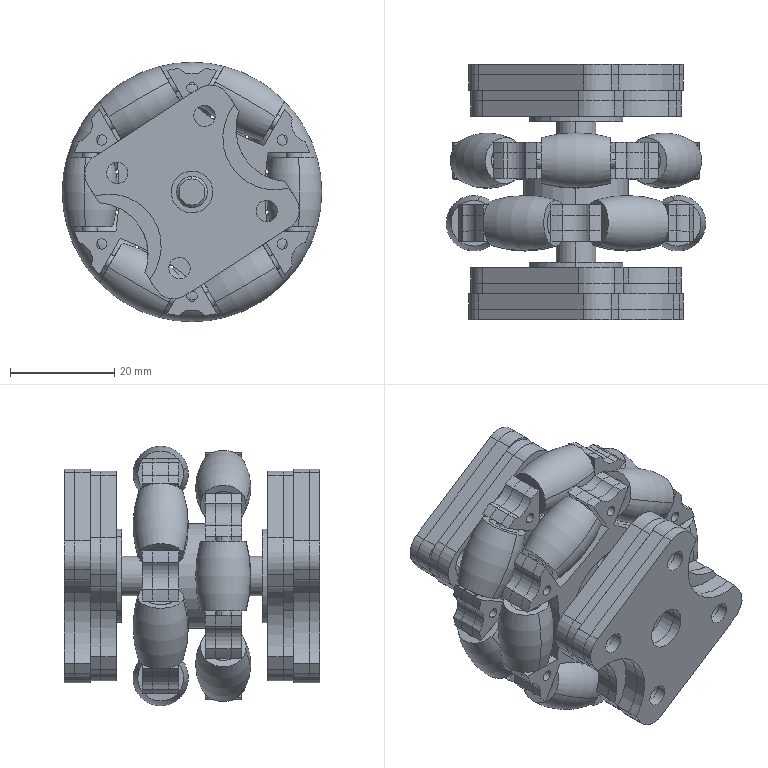Assembly | SolidWorks | mm | 41 component files | 41 solids | 908 faces | volume 40987 mm3 | cylinder 540 | plane 336 | torus 24 | cone 8 | commonest cylinder face diameters 2 x72 47.6 x72 6 x56 7 x48 3 x48 96.351 x42 4.2 x32 4.1 x32
Bill of materials:
6 15 5 F | 2 |  | Flanged bushing-like shape: a thin circular flange joined to a shorter-diameter cylindrical hub on one side, with a single central through bore.
FrontWheelAxis | 1 | 6061 Alloy | Turned shaft with a central circular flange. The flange has four equally spaced axial through holes, and the shaft steps down in diameter on each side to smaller end journals.
FrontWheelBearingPlate | 2 |  | Flat plate with a roughly rhombic/diamond outline, two opposite concave arc-shaped edge cutouts, a large central round hole, and four corner holes that appear counterbored.
FrontWheelPadPlate | 2 |  | Flat plate with the same outline as the previous variant: diamond-like shape with rounded corners, two opposite concave arc cutouts, a large central round hole and four plain corner through holes.
FrontWheelSidePadPlate | 2 |  | Thin flat plate with rounded corners and two deep opposite concave arc cutouts. It has a medium-size central round hole and four smaller holes near the corners.
FrontWheelSideThickPlate | 2 |  | Flat plate with rounded corners, two deep opposite concave arc cutouts, a central round hole and four plain corner holes. The outline appears to match unnamed part but the plate is thicker.
Axis | 12 | Copper | Stepped cylindrical pin: a longer large-diameter central body with a short, smaller-diameter coaxial stub at each end.
MiddleChip | 2 | 1060 Alloy | Thin flat plate with a hexagon-like centre that has concave sides, six radial arms, a large central hole and four smaller holes around it. Each arm tip has a small hole and a concave arc end with notched side features.
Roller | 12 | Rubber | Hollow barrel-shaped sleeve: the outer surface bulges outward and is largest at mid-length, with a straight cylindrical through bore and flat annular end faces.
SidePlate | 4 | 1060 Alloy | Thin flat ring-like plate with a large central circular opening, a hexagon-like outer web with concave sides, and six triangular radial arms, each with a small hole and a concave arc at the tip.
Mates:
1. concentric | FrontWheelAxis-1 face at (0.3183, -9.6, 37) dir (0, 1, 0) r 3.8 | Half-1/MiddleChip-1 face at (0.3183, -0.6003, 37) dir (0, -1, 0) r 4
2. coincident | FrontWheelAxis-1 face at (0.3183, -0.6003, 37) dir (0, -1, 0) | Half-1/MiddleChip-1 face at (-16.727, -0.6003, 48.144) dir (0, 1, 0)
3. concentric | FrontWheelAxis-1 face at (-6.682, 8.4, 37) dir (0, -1, 0) r 1.2 | Half-1/MiddleChip-1 face at (-6.682, -0.6003, 37) dir (0, -1, 0) r 1.6
4. concentric | FrontWheelAxis-1 face at (0.3183, 17.4, 37) dir (0, -1, 0) r 3.8 | Half-2/MiddleChip-1 face at (0.3183, 11.4, 37) dir (0, -1, 0) r 4
5. coincident | FrontWheelAxis-1 face at (0.3183, 8.4, 37) dir (0, 1, 0) | Half-2/MiddleChip-1 face at (-10.825, 8.4, 19.954) dir (0, -1, 0)
6. concentric | FrontWheelAxis-1 face at (-6.682, 8.4, 37) dir (0, -1, 0) r 1.2 | Half-2/MiddleChip-1 face at (-6.682, 11.4, 37) dir (0, -1, 0) r 1.6
7. concentric | FrontWheelAxis-1 face at (0.3183, 22.4, 37) dir (0, -1, 0) r 3 | 6 15 5 F-1 face at (0.3183, 17.4, 37) dir (0, 1, 0) r 3
8. coincident | FrontWheelAxis-1 face at (0.3183, 17.4, 37) dir (0, 1, 0) | 6 15 5 F-1 face at (0.3183, 17.4, 37) dir (0, -1, 0)
9. concentric | FrontWheelAxis-1 face at (0.3183, -14.6, 37) dir (0, 1, 0) r 3 | 6 15 5 F-2 face at (0.3183, -9.6, 37) dir (0, -1, 0) r 7.5
10. coincident | FrontWheelAxis-1 face at (0.3183, -9.6, 37) dir (0, -1, 0) | 6 15 5 F-2 face at (0.3183, -9.6, 37) dir (0, 1, 0)
11. concentric | 6 15 5 F-1 face at (0.3183, 17.4, 37) dir (0, 1, 0) r 7.5 | FrontWheelBearingPlate-1 face at (0.3183, 18.4, 37) dir (0, 1, 0) r 7.5
12. coincident | 6 15 5 F-1 face at (0.3183, 18.4, 37) dir (0, 1, 0) | FrontWheelBearingPlate-1 face at (0.3183, 18.4, 37) dir (0, -1, 0)
13. concentric | 6 15 5 F-2 face at (0.3183, -9.6, 37) dir (0, -1, 0) r 7.5 | FrontWheelBearingPlate-2 face at (0.3183, -10.6, 37) dir (0, -1, 0) r 7.5
14. coincident | 6 15 5 F-2 face at (0.3183, -10.6, 37) dir (0, -1, 0) | FrontWheelBearingPlate-2 face at (0.3183, -10.6, 37) dir (0, 1, 0)
15. coincident | FrontWheelBearingPlate-1 face at (-4.38, 18.4, 14.938) dir (0.5469, 0, -0.8372) | FrontWheelBearingPlate-2 face at (22.409, -10.6, 32.44) dir (0.5469, 0, -0.8372)
16. concentric | 6 15 5 F-1 face at (0.3183, 17.4, 37) dir (0, 1, 0) r 7.5 | FrontWheelPadPlate-1 face at (0.3183, 23.4, 37) dir (0, -1, 0) r 7.5
17. concentric | FrontWheelBearingPlate-1 face at (14.652, 18.4, 33.344) dir (0, 1, 0) r 2.1 | FrontWheelPadPlate-1 face at (14.652, 23.4, 33.344) dir (0, -1, 0) r 2.1
18. coincident | FrontWheelBearingPlate-1 face at (0.3183, 21.4, 37) dir (0, 1, 0) | FrontWheelPadPlate-1 face at (0.3183, 21.4, 37) dir (0, -1, 0)
19. concentric | 6 15 5 F-2 face at (0.3183, -9.6, 37) dir (0, -1, 0) r 7.5 | FrontWheelPadPlate-2 face at (0.3183, -13.6, 37) dir (0, -1, 0) r 7.5
20. concentric | FrontWheelBearingPlate-2 face at (14.652, -10.6, 33.344) dir (0, -1, 0) r 2.1 | FrontWheelPadPlate-2 face at (14.652, -13.6, 33.344) dir (0, -1, 0) r 2.1
21. coincident | FrontWheelBearingPlate-2 face at (0.3183, -13.6, 37) dir (0, -1, 0) | FrontWheelPadPlate-2 face at (0.3183, -13.6, 37) dir (0, 1, 0)
22. concentric | FrontWheelPadPlate-1 face at (0.3183, 23.4, 37) dir (0, -1, 0) r 7.5 | FrontWheelSideThickPlate-2 face at (0.3183, 23.4, 37) dir (0, 1, 0) r 4
23. concentric | FrontWheelPadPlate-1 face at (14.652, 23.4, 33.344) dir (0, -1, 0) r 2.1 | FrontWheelSideThickPlate-2 face at (14.652, 23.4, 33.344) dir (0, 1, 0) r 2.05
24. coincident | FrontWheelPadPlate-1 face at (0.3183, 23.4, 37) dir (0, 1, 0) | FrontWheelSideThickPlate-2 face at (0.3183, 23.4, 37) dir (0, -1, 0)
25. concentric | FrontWheelSidePadPlate-1 face at (0.3183, 28.4, 37) dir (0, -1, 0) r 4 | FrontWheelSideThickPlate-2 face at (0.3183, 23.4, 37) dir (0, 1, 0) r 4
26. concentric | FrontWheelSidePadPlate-1 face at (14.652, 28.4, 33.344) dir (0, -1, 0) r 2.05 | FrontWheelSideThickPlate-2 face at (14.652, 23.4, 33.344) dir (0, 1, 0) r 2.05
27. coincident | FrontWheelSidePadPlate-1 face at (0.3183, 26.4, 37) dir (0, -1, 0) | FrontWheelSideThickPlate-2 face at (0.3183, 26.4, 37) dir (0, 1, 0)
28. concentric | FrontWheelPadPlate-2 face at (0.3183, -13.6, 37) dir (0, -1, 0) r 7.5 | FrontWheelSideThickPlate-1 face at (0.3183, -18.6, 37) dir (0, 1, 0) r 4
29. concentric | FrontWheelPadPlate-2 face at (14.652, -13.6, 33.344) dir (0, -1, 0) r 2.1 | FrontWheelSideThickPlate-1 face at (14.652, -18.6, 33.344) dir (0, 1, 0) r 2.05
30. coincident | FrontWheelPadPlate-2 face at (0.3183, -15.6, 37) dir (0, -1, 0) | FrontWheelSideThickPlate-1 face at (0.3183, -15.6, 37) dir (0, 1, 0)
31. concentric | FrontWheelSidePadPlate-2 face at (0.3183, -18.6, 37) dir (0, -1, 0) r 4 | FrontWheelSideThickPlate-1 face at (0.3183, -18.6, 37) dir (0, 1, 0) r 4
32. coincident | FrontWheelSidePadPlate-2 face at (0.3183, -18.6, 37) dir (0, 1, 0) | FrontWheelSideThickPlate-1 face at (0.3183, -18.6, 37) dir (0, -1, 0)
33. concentric | FrontWheelSidePadPlate-2 face at (14.652, -18.6, 33.344) dir (0, -1, 0) r 2.05 | FrontWheelSideThickPlate-1 face at (14.652, -18.6, 33.344) dir (0, 1, 0) r 2.05
34. concentric | MiddleChip-1 face at (0, 3.051, 49.337) dir (0, 0, -1) r 4 | SidePlate-1 face at (0, 3.051, 51.337) dir (0, 0, -1) r 10.5
35. concentric | MiddleChip-1 face at (-17.321, 13.051, 49.337) dir (0, 0, -1) r 1 | SidePlate-1 face at (-17.321, 13.051, 51.337) dir (0, 0, -1) r 1
36. coincident | MiddleChip-1 face at (-17.046, -8.093, 49.337) dir (0, 0, 1) | SidePlate-1 face at (0, 3.051, 49.337) dir (0, 0, -1)
37. coincident | MiddleChip-1 face at (-17.046, -8.093, 46.337) dir (0, 0, -1) | SidePlate-2 face at (0, 3.051, 46.337) dir (0, 0, 1)
38. concentric | MiddleChip-1 face at (0, 3.051, 49.337) dir (0, 0, -1) r 4 | SidePlate-2 face at (0, 3.051, 46.337) dir (0, 0, -1) r 10.5
39. concentric | MiddleChip-1 face at (-17.321, 13.051, 49.337) dir (0, 0, -1) r 1 | SidePlate-2 face at (-17.321, 13.051, 46.337) dir (0, 0, -1) r 1
40. concentric | Axis-1 face at (-15.596, 16.664, 47.837) dir (0.866, 0.5, 0) r 3 | Roller-1 face at (-3.991, 23.364, 47.837) dir (-0.866, -0.5, 0) r 3
41. coincident | Axis-1 face at (-15.596, 16.664, 47.837) dir (-0.866, -0.5, 0) | Roller-1 face at (-17.605, 20.143, 28.142) dir (-0.866, -0.5, 0)
42. tangent | SidePlate-2 face at (0, 3.051, 46.337) dir (0, 0, 1) | Axis-1 face at (-17.588, 15.514, 47.837) dir (0.866, 0.5, 0) r 1.5
43. tangent | MiddleChip-1 face at (-28.153, 11.146, 49.337) dir (0.5, -0.866, 0) | Axis-1 face at (-17.588, 15.514, 47.837) dir (0.866, 0.5, 0) r 1.5
44. coincident | MiddleChip-1 face at (-7.23, -2.426, 49.337) dir (0.866, 0.5, 0) | Axis-1 face at (-17.588, 15.514, 47.837) dir (-0.866, -0.5, 0)
45. coincident | MiddleChip-1 face at (-7.23, -2.426, 49.337) dir (0.866, 0.5, 0) | Axis-1 face at (-17.588, 15.514, 47.837) dir (-0.866, -0.5, 0)